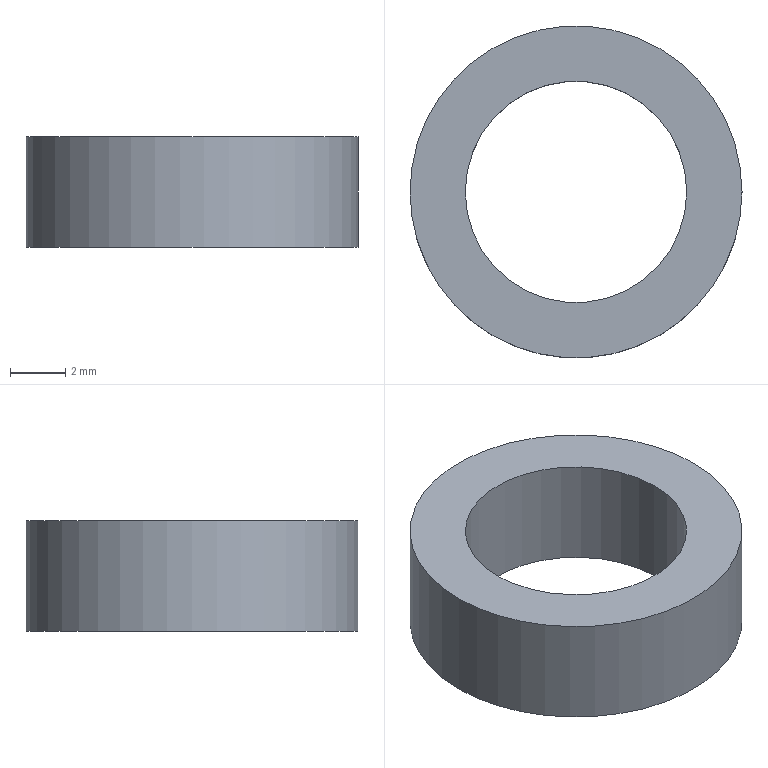Component | NX | PACKING | 1 solid | 4 faces | box 12 x 12 x 4 mm | volume 251 mm3 | cylinder 2 | plane 2 | commonest cylinder face diameters 12 x1 8 x1
STEP:
#1=CARTESIAN_POINT('',(0.,0.,0.));
#2=DIRECTION('',(0.,0.,1.));
#3=DIRECTION('',(1.,0.,0.));
#4=AXIS2_PLACEMENT_3D('',#1,#2,#3);
#5=CARTESIAN_POINT('',(6.,14.,43.7));
#6=VERTEX_POINT('',#5);
#7=CARTESIAN_POINT('',(-0.,14.,43.7));
#8=DIRECTION('',(0.,0.,1.));
#9=DIRECTION('',(1.,0.,0.));
#10=AXIS2_PLACEMENT_3D('',#7,#8,#9);
#11=CIRCLE('',#10,6.);
#12=CARTESIAN_POINT('',(-0.,14.,43.7));
#13=DIRECTION('',(0.,0.,-1.));
#14=DIRECTION('',(-1.,0.,0.));
#15=AXIS2_PLACEMENT_3D('',#12,#13,#14);
#16=CYLINDRICAL_SURFACE('',#15,6.);
#17=CARTESIAN_POINT('',(9.425,0.));
#18=DIRECTION('',(-1.,0.));
#19=VECTOR('',#18,1.);
#20=LINE('',#17,#19);
#21=(GEOMETRIC_REPRESENTATION_CONTEXT(2)PARAMETRIC_REPRESENTATION_CONTEXT()REPRESENTATION_CONTEXT('',''));
#22=DEFINITIONAL_REPRESENTATION('',(#20),#21);
#23=PCURVE('',#16,#22);
#24=CARTESIAN_POINT('',(-0.,14.,43.7));
#25=DIRECTION('',(0.,0.,1.));
#26=DIRECTION('',(1.,0.,0.));
#27=AXIS2_PLACEMENT_3D('',#24,#25,#26);
#28=PLANE('',#27);
#29=CARTESIAN_POINT('',(0.,0.));
#30=DIRECTION('',(1.,0.));
#31=AXIS2_PLACEMENT_2D('',#29,#30);
#32=CIRCLE('',#31,6.);
#33=(GEOMETRIC_REPRESENTATION_CONTEXT(2)PARAMETRIC_REPRESENTATION_CONTEXT()REPRESENTATION_CONTEXT('',''));
#34=DEFINITIONAL_REPRESENTATION('',(#32),#33);
#35=PCURVE('',#28,#34);
#36=SURFACE_CURVE('',#11,(#23,#35),.PCURVE_S1.);
#37=EDGE_CURVE('',#6,#6,#36,.T.);
#38=ORIENTED_EDGE('',*,*,#37,.F.);
#39=CARTESIAN_POINT('',(6.,14.,39.7));
#40=VERTEX_POINT('',#39);
#41=CARTESIAN_POINT('',(6.,14.,43.7));
#42=CARTESIAN_POINT('',(6.,14.,39.7));
#43=B_SPLINE_CURVE_WITH_KNOTS('',1,(#41,#42),.UNSPECIFIED.,.F.,.F.,(2,2),(0.,4.),.PIECEWISE_BEZIER_KNOTS.);
#44=CARTESIAN_POINT('',(9.425,0.));
#45=DIRECTION('',(0.,1.));
#46=VECTOR('',#45,1.);
#47=LINE('',#44,#46);
#48=(GEOMETRIC_REPRESENTATION_CONTEXT(2)PARAMETRIC_REPRESENTATION_CONTEXT()REPRESENTATION_CONTEXT('',''));
#49=DEFINITIONAL_REPRESENTATION('',(#47),#48);
#50=PCURVE('',#16,#49);
#51=CARTESIAN_POINT('',(3.142,0.));
#52=DIRECTION('',(0.,1.));
#53=VECTOR('',#52,1.);
#54=LINE('',#51,#53);
#55=(GEOMETRIC_REPRESENTATION_CONTEXT(2)PARAMETRIC_REPRESENTATION_CONTEXT()REPRESENTATION_CONTEXT('',''));
#56=DEFINITIONAL_REPRESENTATION('',(#54),#55);
#57=PCURVE('',#16,#56);
#58=SEAM_CURVE('',#43,(#50,#57),.PCURVE_S1.);
#59=EDGE_CURVE('',#6,#40,#58,.T.);
#60=ORIENTED_EDGE('',*,*,#59,.T.);
#61=CARTESIAN_POINT('',(-0.,14.,39.7));
#62=DIRECTION('',(0.,0.,1.));
#63=DIRECTION('',(1.,0.,0.));
#64=AXIS2_PLACEMENT_3D('',#61,#62,#63);
#65=CIRCLE('',#64,6.);
#66=CARTESIAN_POINT('',(9.425,4.));
#67=DIRECTION('',(-1.,0.));
#68=VECTOR('',#67,1.);
#69=LINE('',#66,#68);
#70=(GEOMETRIC_REPRESENTATION_CONTEXT(2)PARAMETRIC_REPRESENTATION_CONTEXT()REPRESENTATION_CONTEXT('',''));
#71=DEFINITIONAL_REPRESENTATION('',(#69),#70);
#72=PCURVE('',#16,#71);
#73=CARTESIAN_POINT('',(-0.,14.,39.7));
#74=DIRECTION('',(0.,0.,1.));
#75=DIRECTION('',(1.,0.,0.));
#76=AXIS2_PLACEMENT_3D('',#73,#74,#75);
#77=PLANE('',#76);
#78=CARTESIAN_POINT('',(0.,0.));
#79=DIRECTION('',(1.,0.));
#80=AXIS2_PLACEMENT_2D('',#78,#79);
#81=CIRCLE('',#80,6.);
#82=(GEOMETRIC_REPRESENTATION_CONTEXT(2)PARAMETRIC_REPRESENTATION_CONTEXT()REPRESENTATION_CONTEXT('',''));
#83=DEFINITIONAL_REPRESENTATION('',(#81),#82);
#84=PCURVE('',#77,#83);
#85=SURFACE_CURVE('',#65,(#72,#84),.PCURVE_S1.);
#86=EDGE_CURVE('',#40,#40,#85,.T.);
#87=ORIENTED_EDGE('',*,*,#86,.T.);
#88=ORIENTED_EDGE('',*,*,#59,.F.);
#89=EDGE_LOOP('',(#38,#60,#87,#88));
#90=FACE_BOUND('',#89,.T.);
#91=ADVANCED_FACE('',(#90),#16,.T.);
#92=CARTESIAN_POINT('',(4.,14.,43.7));
#93=VERTEX_POINT('',#92);
#94=CARTESIAN_POINT('',(-0.,14.,43.7));
#95=DIRECTION('',(0.,0.,1.));
#96=DIRECTION('',(1.,0.,0.));
#97=AXIS2_PLACEMENT_3D('',#94,#95,#96);
#98=CIRCLE('',#97,4.);
#99=CARTESIAN_POINT('',(-0.,14.,43.7));
#100=DIRECTION('',(0.,0.,-1.));
#101=DIRECTION('',(-1.,0.,0.));
#102=AXIS2_PLACEMENT_3D('',#99,#100,#101);
#103=CYLINDRICAL_SURFACE('',#102,4.);
#104=CARTESIAN_POINT('',(9.425,0.));
#105=DIRECTION('',(-1.,0.));
#106=VECTOR('',#105,1.);
#107=LINE('',#104,#106);
#108=(GEOMETRIC_REPRESENTATION_CONTEXT(2)PARAMETRIC_REPRESENTATION_CONTEXT()REPRESENTATION_CONTEXT('',''));
#109=DEFINITIONAL_REPRESENTATION('',(#107),#108);
#110=PCURVE('',#103,#109);
#111=CARTESIAN_POINT('',(0.,0.));
#112=DIRECTION('',(1.,0.));
#113=AXIS2_PLACEMENT_2D('',#111,#112);
#114=CIRCLE('',#113,4.);
#115=(GEOMETRIC_REPRESENTATION_CONTEXT(2)PARAMETRIC_REPRESENTATION_CONTEXT()REPRESENTATION_CONTEXT('',''));
#116=DEFINITIONAL_REPRESENTATION('',(#114),#115);
#117=PCURVE('',#28,#116);
#118=SURFACE_CURVE('',#98,(#110,#117),.PCURVE_S1.);
#119=EDGE_CURVE('',#93,#93,#118,.T.);
#120=ORIENTED_EDGE('',*,*,#119,.F.);
#121=CARTESIAN_POINT('',(4.,14.,39.7));
#122=VERTEX_POINT('',#121);
#123=CARTESIAN_POINT('',(4.,14.,43.7));
#124=CARTESIAN_POINT('',(4.,14.,39.7));
#125=B_SPLINE_CURVE_WITH_KNOTS('',1,(#123,#124),.UNSPECIFIED.,.F.,.F.,(2,2),(0.,4.),.PIECEWISE_BEZIER_KNOTS.);
#126=CARTESIAN_POINT('',(9.425,0.));
#127=DIRECTION('',(0.,1.));
#128=VECTOR('',#127,1.);
#129=LINE('',#126,#128);
#130=(GEOMETRIC_REPRESENTATION_CONTEXT(2)PARAMETRIC_REPRESENTATION_CONTEXT()REPRESENTATION_CONTEXT('',''));
#131=DEFINITIONAL_REPRESENTATION('',(#129),#130);
#132=PCURVE('',#103,#131);
#133=CARTESIAN_POINT('',(3.142,0.));
#134=DIRECTION('',(0.,1.));
#135=VECTOR('',#134,1.);
#136=LINE('',#133,#135);
#137=(GEOMETRIC_REPRESENTATION_CONTEXT(2)PARAMETRIC_REPRESENTATION_CONTEXT()REPRESENTATION_CONTEXT('',''));
#138=DEFINITIONAL_REPRESENTATION('',(#136),#137);
#139=PCURVE('',#103,#138);
#140=SEAM_CURVE('',#125,(#132,#139),.PCURVE_S1.);
#141=EDGE_CURVE('',#93,#122,#140,.T.);
#142=ORIENTED_EDGE('',*,*,#141,.T.);
#143=CARTESIAN_POINT('',(-0.,14.,39.7));
#144=DIRECTION('',(0.,0.,1.));
#145=DIRECTION('',(1.,0.,0.));
#146=AXIS2_PLACEMENT_3D('',#143,#144,#145);
#147=CIRCLE('',#146,4.);
#148=CARTESIAN_POINT('',(9.425,4.));
#149=DIRECTION('',(-1.,0.));
#150=VECTOR('',#149,1.);
#151=LINE('',#148,#150);
#152=(GEOMETRIC_REPRESENTATION_CONTEXT(2)PARAMETRIC_REPRESENTATION_CONTEXT()REPRESENTATION_CONTEXT('',''));
#153=DEFINITIONAL_REPRESENTATION('',(#151),#152);
#154=PCURVE('',#103,#153);
#155=CARTESIAN_POINT('',(0.,0.));
#156=DIRECTION('',(1.,0.));
#157=AXIS2_PLACEMENT_2D('',#155,#156);
#158=CIRCLE('',#157,4.);
#159=(GEOMETRIC_REPRESENTATION_CONTEXT(2)PARAMETRIC_REPRESENTATION_CONTEXT()REPRESENTATION_CONTEXT('',''));
#160=DEFINITIONAL_REPRESENTATION('',(#158),#159);
#161=PCURVE('',#77,#160);
#162=SURFACE_CURVE('',#147,(#154,#161),.PCURVE_S1.);
#163=EDGE_CURVE('',#122,#122,#162,.T.);
#164=ORIENTED_EDGE('',*,*,#163,.T.);
#165=ORIENTED_EDGE('',*,*,#141,.F.);
#166=EDGE_LOOP('',(#120,#142,#164,#165));
#167=FACE_BOUND('',#166,.F.);
#168=ADVANCED_FACE('',(#167),#103,.F.);
#169=ORIENTED_EDGE('',*,*,#37,.T.);
#170=EDGE_LOOP('',(#169));
#171=FACE_BOUND('',#170,.T.);
#172=ORIENTED_EDGE('',*,*,#119,.F.);
#173=EDGE_LOOP('',(#172));
#174=FACE_BOUND('',#173,.T.);
#175=ADVANCED_FACE('',(#171,#174),#28,.T.);
#176=ORIENTED_EDGE('',*,*,#86,.F.);
#177=EDGE_LOOP('',(#176));
#178=FACE_BOUND('',#177,.T.);
#179=ORIENTED_EDGE('',*,*,#163,.T.);
#180=EDGE_LOOP('',(#179));
#181=FACE_BOUND('',#180,.T.);
#182=ADVANCED_FACE('',(#178,#181),#77,.F.);
#183=CLOSED_SHELL('',(#91,#168,#175,#182));
#184=MANIFOLD_SOLID_BREP('',#183);
#185=(LENGTH_UNIT()NAMED_UNIT(*)SI_UNIT(.MILLI.,.METRE.));
#186=UNCERTAINTY_MEASURE_WITH_UNIT(LENGTH_MEASURE(0.00001),#185,'','');
#187=(NAMED_UNIT(*)PLANE_ANGLE_UNIT()SI_UNIT($,.RADIAN.));
#188=(NAMED_UNIT(*)SI_UNIT($,.STERADIAN.)SOLID_ANGLE_UNIT());
#189=(GEOMETRIC_REPRESENTATION_CONTEXT(3)GLOBAL_UNCERTAINTY_ASSIGNED_CONTEXT((#186))GLOBAL_UNIT_ASSIGNED_CONTEXT((#185,#187,#188))REPRESENTATION_CONTEXT('',''));
#190=ADVANCED_BREP_SHAPE_REPRESENTATION('',(#4,#184),#189);